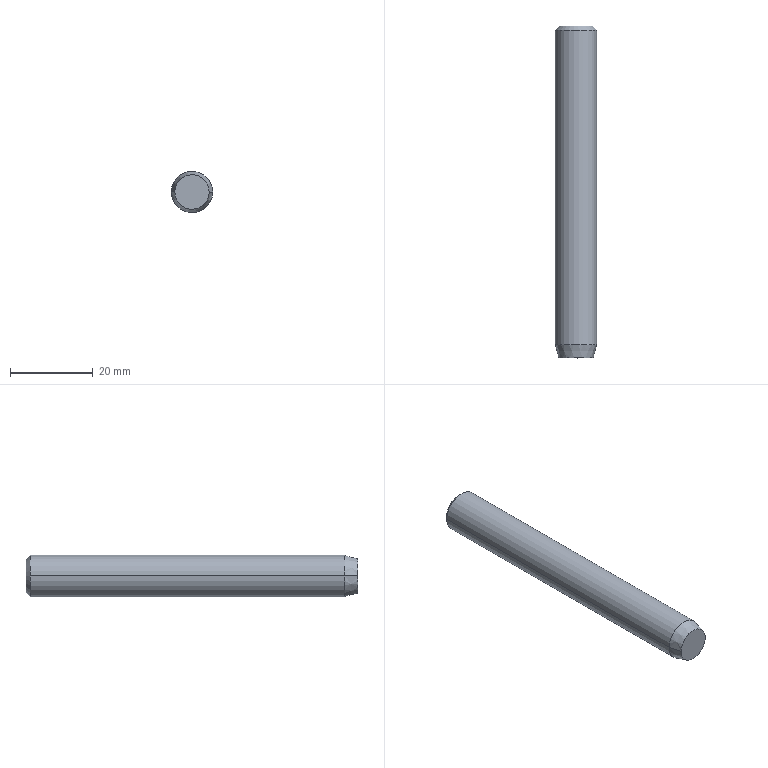Component | SolidWorks | GB_T15389-1994ScrewM10_100-1 | 1 solid | 8 faces | box 10 x 80 x 10 mm | volume 6227 mm3 | cone 4 | cylinder 2 | plane 2 | commonest cylinder face diameters 10 x2
STEP:
#1=COLOUR_RGB('',0.7922,0.8196,0.9333);
#2=FILL_AREA_STYLE_COLOUR('',#1);
#3=FILL_AREA_STYLE('',(#2));
#4=SURFACE_STYLE_FILL_AREA(#3);
#5=SURFACE_SIDE_STYLE('',(#4));
#6=SURFACE_STYLE_USAGE(.BOTH.,#5);
#7=PRESENTATION_STYLE_ASSIGNMENT((#6));
#8=CARTESIAN_POINT('',(3.617,6.768,0.0009758));
#9=VERTEX_POINT('',#8);
#10=CARTESIAN_POINT('',(3.942,6.768,-0.0009758));
#11=VERTEX_POINT('',#10);
#12=CARTESIAN_POINT('',(3.78,6.768,0.));
#13=DIRECTION('',(0.,-1.,-0.));
#14=DIRECTION('',(1.,0.,-0.005996));
#15=AXIS2_PLACEMENT_3D('',#12,#13,#14);
#16=CIRCLE('',#15,0.1628);
#17=EDGE_CURVE('',#9,#11,#16,.T.);
#18=ORIENTED_EDGE('',*,*,#17,.F.);
#19=CARTESIAN_POINT('',(3.583,6.895,0.00118));
#20=VERTEX_POINT('',#19);
#21=CARTESIAN_POINT('',(3.583,6.895,0.00118));
#22=DIRECTION('',(-0.2588,0.9659,0.001552));
#23=VECTOR('',#22,39.37);
#24=LINE('',#21,#23);
#25=EDGE_CURVE('',#9,#20,#24,.T.);
#26=ORIENTED_EDGE('',*,*,#25,.T.);
#27=CARTESIAN_POINT('',(3.976,6.895,-0.00118));
#28=VERTEX_POINT('',#27);
#29=CARTESIAN_POINT('',(3.78,6.895,0.));
#30=DIRECTION('',(-0.,1.,0.));
#31=DIRECTION('',(-1.,0.,0.005996));
#32=AXIS2_PLACEMENT_3D('',#29,#30,#31);
#33=CIRCLE('',#32,0.1969);
#34=EDGE_CURVE('',#28,#20,#33,.T.);
#35=ORIENTED_EDGE('',*,*,#34,.F.);
#36=CARTESIAN_POINT('',(3.976,6.895,-0.00118));
#37=DIRECTION('',(0.2588,0.9659,-0.001552));
#38=VECTOR('',#37,39.37);
#39=LINE('',#36,#38);
#40=EDGE_CURVE('',#11,#28,#39,.T.);
#41=ORIENTED_EDGE('',*,*,#40,.F.);
#42=EDGE_LOOP('',(#18,#26,#35,#41));
#43=FACE_OUTER_BOUND('',#42,.T.);
#44=CARTESIAN_POINT('',(3.78,6.895,0.));
#45=DIRECTION('',(-0.,1.,0.));
#46=DIRECTION('',(1.,0.,-0.005996));
#47=AXIS2_PLACEMENT_3D('',#44,#45,#46);
#48=CONICAL_SURFACE('',#47,0.1969,0.2618);
#49=ADVANCED_FACE('',(#43),#48,.T.);
#50=CARTESIAN_POINT('',(3.937,9.917,-0.0009442));
#51=VERTEX_POINT('',#50);
#52=CARTESIAN_POINT('',(3.622,9.917,0.0009442));
#53=VERTEX_POINT('',#52);
#54=CARTESIAN_POINT('',(3.78,9.917,0.));
#55=DIRECTION('',(-0.,1.,0.));
#56=DIRECTION('',(1.,0.,-0.005996));
#57=AXIS2_PLACEMENT_3D('',#54,#55,#56);
#58=CIRCLE('',#57,0.1575);
#59=EDGE_CURVE('',#51,#53,#58,.T.);
#60=ORIENTED_EDGE('',*,*,#59,.F.);
#61=CARTESIAN_POINT('',(3.976,9.878,-0.00118));
#62=VERTEX_POINT('',#61);
#63=CARTESIAN_POINT('',(3.937,9.917,-0.0009442));
#64=DIRECTION('',(0.7071,-0.7071,-0.004239));
#65=VECTOR('',#64,39.37);
#66=LINE('',#63,#65);
#67=EDGE_CURVE('',#51,#62,#66,.T.);
#68=ORIENTED_EDGE('',*,*,#67,.T.);
#69=CARTESIAN_POINT('',(3.583,9.878,0.00118));
#70=VERTEX_POINT('',#69);
#71=CARTESIAN_POINT('',(3.78,9.878,0.));
#72=DIRECTION('',(0.,-1.,-0.));
#73=DIRECTION('',(1.,0.,-0.005996));
#74=AXIS2_PLACEMENT_3D('',#71,#72,#73);
#75=CIRCLE('',#74,0.1969);
#76=EDGE_CURVE('',#70,#62,#75,.T.);
#77=ORIENTED_EDGE('',*,*,#76,.F.);
#78=CARTESIAN_POINT('',(3.622,9.917,0.0009442));
#79=DIRECTION('',(-0.7071,-0.7071,0.004239));
#80=VECTOR('',#79,39.37);
#81=LINE('',#78,#80);
#82=EDGE_CURVE('',#53,#70,#81,.T.);
#83=ORIENTED_EDGE('',*,*,#82,.F.);
#84=EDGE_LOOP('',(#60,#68,#77,#83));
#85=FACE_OUTER_BOUND('',#84,.T.);
#86=CARTESIAN_POINT('',(3.78,9.917,0.));
#87=DIRECTION('',(0.,-1.,-0.));
#88=DIRECTION('',(-1.,0.,0.005996));
#89=AXIS2_PLACEMENT_3D('',#86,#87,#88);
#90=CONICAL_SURFACE('',#89,0.1575,0.7854);
#91=ADVANCED_FACE('',(#85),#90,.T.);
#92=ORIENTED_EDGE('',*,*,#34,.T.);
#93=CARTESIAN_POINT('',(3.583,6.768,0.00118));
#94=DIRECTION('',(-0.,1.,0.));
#95=VECTOR('',#94,39.37);
#96=LINE('',#93,#95);
#97=EDGE_CURVE('',#20,#70,#96,.T.);
#98=ORIENTED_EDGE('',*,*,#97,.T.);
#99=ORIENTED_EDGE('',*,*,#76,.T.);
#100=CARTESIAN_POINT('',(3.976,6.768,-0.00118));
#101=DIRECTION('',(-0.,1.,0.));
#102=VECTOR('',#101,39.37);
#103=LINE('',#100,#102);
#104=EDGE_CURVE('',#28,#62,#103,.T.);
#105=ORIENTED_EDGE('',*,*,#104,.F.);
#106=EDGE_LOOP('',(#92,#98,#99,#105));
#107=FACE_OUTER_BOUND('',#106,.T.);
#108=CARTESIAN_POINT('',(3.78,6.768,0.));
#109=DIRECTION('',(-0.,1.,0.));
#110=DIRECTION('',(1.,0.,-0.005996));
#111=AXIS2_PLACEMENT_3D('',#108,#109,#110);
#112=CYLINDRICAL_SURFACE('',#111,0.1969);
#113=ADVANCED_FACE('',(#107),#112,.T.);
#114=ORIENTED_EDGE('',*,*,#97,.F.);
#115=CARTESIAN_POINT('',(3.78,6.895,0.));
#116=DIRECTION('',(-0.,1.,0.));
#117=DIRECTION('',(-1.,0.,0.005996));
#118=AXIS2_PLACEMENT_3D('',#115,#116,#117);
#119=CIRCLE('',#118,0.1969);
#120=EDGE_CURVE('',#20,#28,#119,.T.);
#121=ORIENTED_EDGE('',*,*,#120,.T.);
#122=ORIENTED_EDGE('',*,*,#104,.T.);
#123=CARTESIAN_POINT('',(3.78,9.878,0.));
#124=DIRECTION('',(0.,-1.,-0.));
#125=DIRECTION('',(1.,0.,-0.005996));
#126=AXIS2_PLACEMENT_3D('',#123,#124,#125);
#127=CIRCLE('',#126,0.1969);
#128=EDGE_CURVE('',#62,#70,#127,.T.);
#129=ORIENTED_EDGE('',*,*,#128,.T.);
#130=EDGE_LOOP('',(#114,#121,#122,#129));
#131=FACE_OUTER_BOUND('',#130,.T.);
#132=CARTESIAN_POINT('',(3.78,6.768,0.));
#133=DIRECTION('',(-0.,1.,0.));
#134=DIRECTION('',(1.,0.,-0.005996));
#135=AXIS2_PLACEMENT_3D('',#132,#133,#134);
#136=CYLINDRICAL_SURFACE('',#135,0.1969);
#137=ADVANCED_FACE('',(#131),#136,.T.);
#138=CARTESIAN_POINT('',(3.78,9.917,0.));
#139=DIRECTION('',(-0.,1.,0.));
#140=DIRECTION('',(1.,0.,-0.005996));
#141=AXIS2_PLACEMENT_3D('',#138,#139,#140);
#142=CIRCLE('',#141,0.1575);
#143=EDGE_CURVE('',#53,#51,#142,.T.);
#144=ORIENTED_EDGE('',*,*,#143,.T.);
#145=ORIENTED_EDGE('',*,*,#59,.T.);
#146=EDGE_LOOP('',(#144,#145));
#147=FACE_OUTER_BOUND('',#146,.T.);
#148=CARTESIAN_POINT('',(3.78,9.917,0.));
#149=DIRECTION('',(-0.,1.,0.));
#150=DIRECTION('',(1.,0.,-0.005996));
#151=AXIS2_PLACEMENT_3D('',#148,#149,#150);
#152=PLANE('',#151);
#153=ADVANCED_FACE('',(#147),#152,.T.);
#154=CARTESIAN_POINT('',(3.78,6.768,0.));
#155=DIRECTION('',(0.,-1.,-0.));
#156=DIRECTION('',(1.,0.,-0.005996));
#157=AXIS2_PLACEMENT_3D('',#154,#155,#156);
#158=CIRCLE('',#157,0.1628);
#159=EDGE_CURVE('',#11,#9,#158,.T.);
#160=ORIENTED_EDGE('',*,*,#159,.T.);
#161=ORIENTED_EDGE('',*,*,#17,.T.);
#162=EDGE_LOOP('',(#160,#161));
#163=FACE_OUTER_BOUND('',#162,.T.);
#164=CARTESIAN_POINT('',(3.78,6.768,0.));
#165=DIRECTION('',(-0.,1.,0.));
#166=DIRECTION('',(1.,0.,-0.005996));
#167=AXIS2_PLACEMENT_3D('',#164,#165,#166);
#168=PLANE('',#167);
#169=ADVANCED_FACE('',(#163),#168,.F.);
#170=ORIENTED_EDGE('',*,*,#67,.F.);
#171=ORIENTED_EDGE('',*,*,#143,.F.);
#172=ORIENTED_EDGE('',*,*,#82,.T.);
#173=ORIENTED_EDGE('',*,*,#128,.F.);
#174=EDGE_LOOP('',(#170,#171,#172,#173));
#175=FACE_OUTER_BOUND('',#174,.T.);
#176=CARTESIAN_POINT('',(3.78,9.917,0.));
#177=DIRECTION('',(0.,-1.,-0.));
#178=DIRECTION('',(-1.,0.,0.005996));
#179=AXIS2_PLACEMENT_3D('',#176,#177,#178);
#180=CONICAL_SURFACE('',#179,0.1575,0.7854);
#181=ADVANCED_FACE('',(#175),#180,.T.);
#182=ORIENTED_EDGE('',*,*,#25,.F.);
#183=ORIENTED_EDGE('',*,*,#159,.F.);
#184=ORIENTED_EDGE('',*,*,#40,.T.);
#185=ORIENTED_EDGE('',*,*,#120,.F.);
#186=EDGE_LOOP('',(#182,#183,#184,#185));
#187=FACE_OUTER_BOUND('',#186,.T.);
#188=CARTESIAN_POINT('',(3.78,6.895,0.));
#189=DIRECTION('',(-0.,1.,0.));
#190=DIRECTION('',(1.,0.,-0.005996));
#191=AXIS2_PLACEMENT_3D('',#188,#189,#190);
#192=CONICAL_SURFACE('',#191,0.1969,0.2618);
#193=ADVANCED_FACE('',(#187),#192,.T.);
#194=CLOSED_SHELL('',(#49,#91,#113,#137,#153,#169,#181,#193));
#195=MANIFOLD_SOLID_BREP('',#194);
#196=STYLED_ITEM('',(#7),#195);
#197=PRESENTATION_LAYER_ASSIGNMENT('','',(#196));
#198=CARTESIAN_POINT('',(0.,0.,0.));
#199=DIRECTION('',(0.,0.,1.));
#200=DIRECTION('',(1.,0.,0.));
#201=AXIS2_PLACEMENT_3D('',#198,#199,#200);
#202=(LENGTH_UNIT()NAMED_UNIT(*)SI_UNIT($,.METRE.));
#203=LENGTH_MEASURE_WITH_UNIT(LENGTH_MEASURE(0.0254),#202);
#204=DIMENSIONAL_EXPONENTS(1.,0.,0.,0.,0.,0.,0.);
#205=(CONVERSION_BASED_UNIT('',#203)LENGTH_UNIT()NAMED_UNIT(#204));
#206=UNCERTAINTY_MEASURE_WITH_UNIT(LENGTH_MEASURE(0.00001),#205,'','');
#207=(NAMED_UNIT(*)PLANE_ANGLE_UNIT()SI_UNIT($,.RADIAN.));
#208=(NAMED_UNIT(*)SI_UNIT($,.STERADIAN.)SOLID_ANGLE_UNIT());
#209=(GEOMETRIC_REPRESENTATION_CONTEXT(3)GLOBAL_UNCERTAINTY_ASSIGNED_CONTEXT((#206))GLOBAL_UNIT_ASSIGNED_CONTEXT((#205,#207,#208))REPRESENTATION_CONTEXT('',''));
#210=ADVANCED_BREP_SHAPE_REPRESENTATION('',(#195,#201),#209);
#211=(LENGTH_UNIT()NAMED_UNIT(*)SI_UNIT($,.METRE.));
#212=LENGTH_MEASURE_WITH_UNIT(LENGTH_MEASURE(0.0254),#211);
#213=DIMENSIONAL_EXPONENTS(1.,0.,0.,0.,0.,0.,0.);
#214=(CONVERSION_BASED_UNIT('',#212)LENGTH_UNIT()NAMED_UNIT(#213));
#215=UNCERTAINTY_MEASURE_WITH_UNIT(LENGTH_MEASURE(0.00001),#214,'','');
#216=(NAMED_UNIT(*)PLANE_ANGLE_UNIT()SI_UNIT($,.RADIAN.));
#217=(NAMED_UNIT(*)SI_UNIT($,.STERADIAN.)SOLID_ANGLE_UNIT());
#218=(GEOMETRIC_REPRESENTATION_CONTEXT(3)GLOBAL_UNCERTAINTY_ASSIGNED_CONTEXT((#215))GLOBAL_UNIT_ASSIGNED_CONTEXT((#214,#216,#217))REPRESENTATION_CONTEXT('',''));
#219=MECHANICAL_DESIGN_GEOMETRIC_PRESENTATION_REPRESENTATION('',(#196),#218);